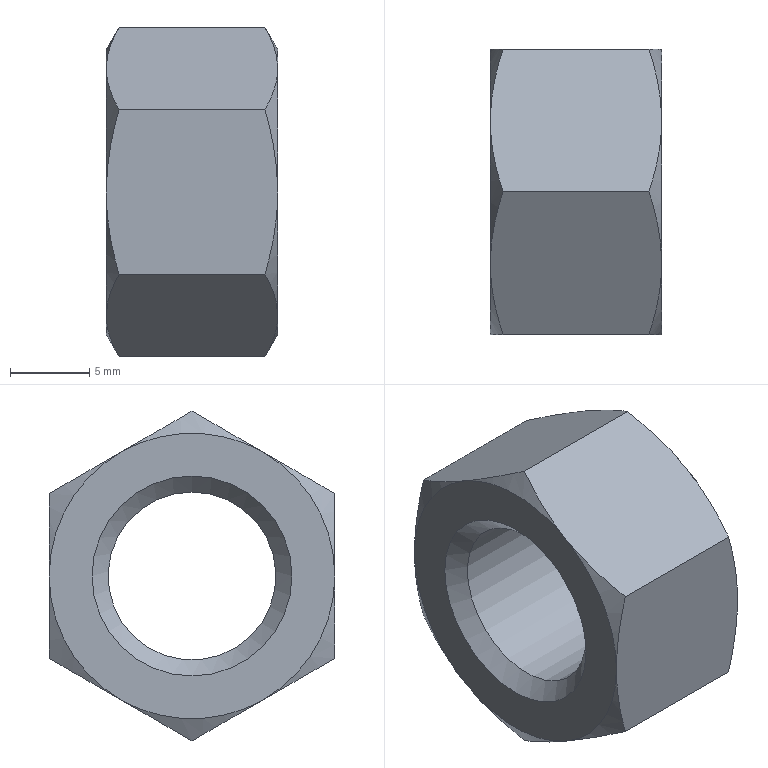Component | NX | GB-T6170_F-2000_M12X1_75 | 1 solid | 23 faces | volume 2032 mm3 | cone 14 | plane 8 | cylinder 1 | commonest cylinder face diameters 10.579 x1